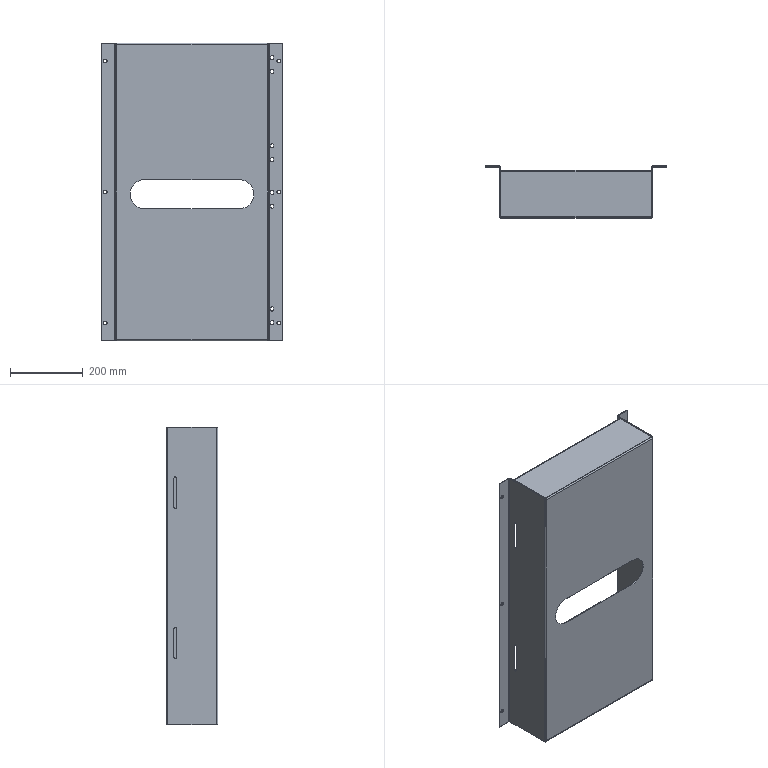Component | SolidWorks | ElectricalCabinetAssembly-1_CabinetAssembly-1_ElectricalCabinet-1 | 1 solid | 137 faces | volume 1368601 mm3 | plane 82 | cylinder 55 | commonest cylinder face diameters 7 x22 10 x12 8 x8 4 x8 80 x3 90 x2 | material Plain Carbon Steel